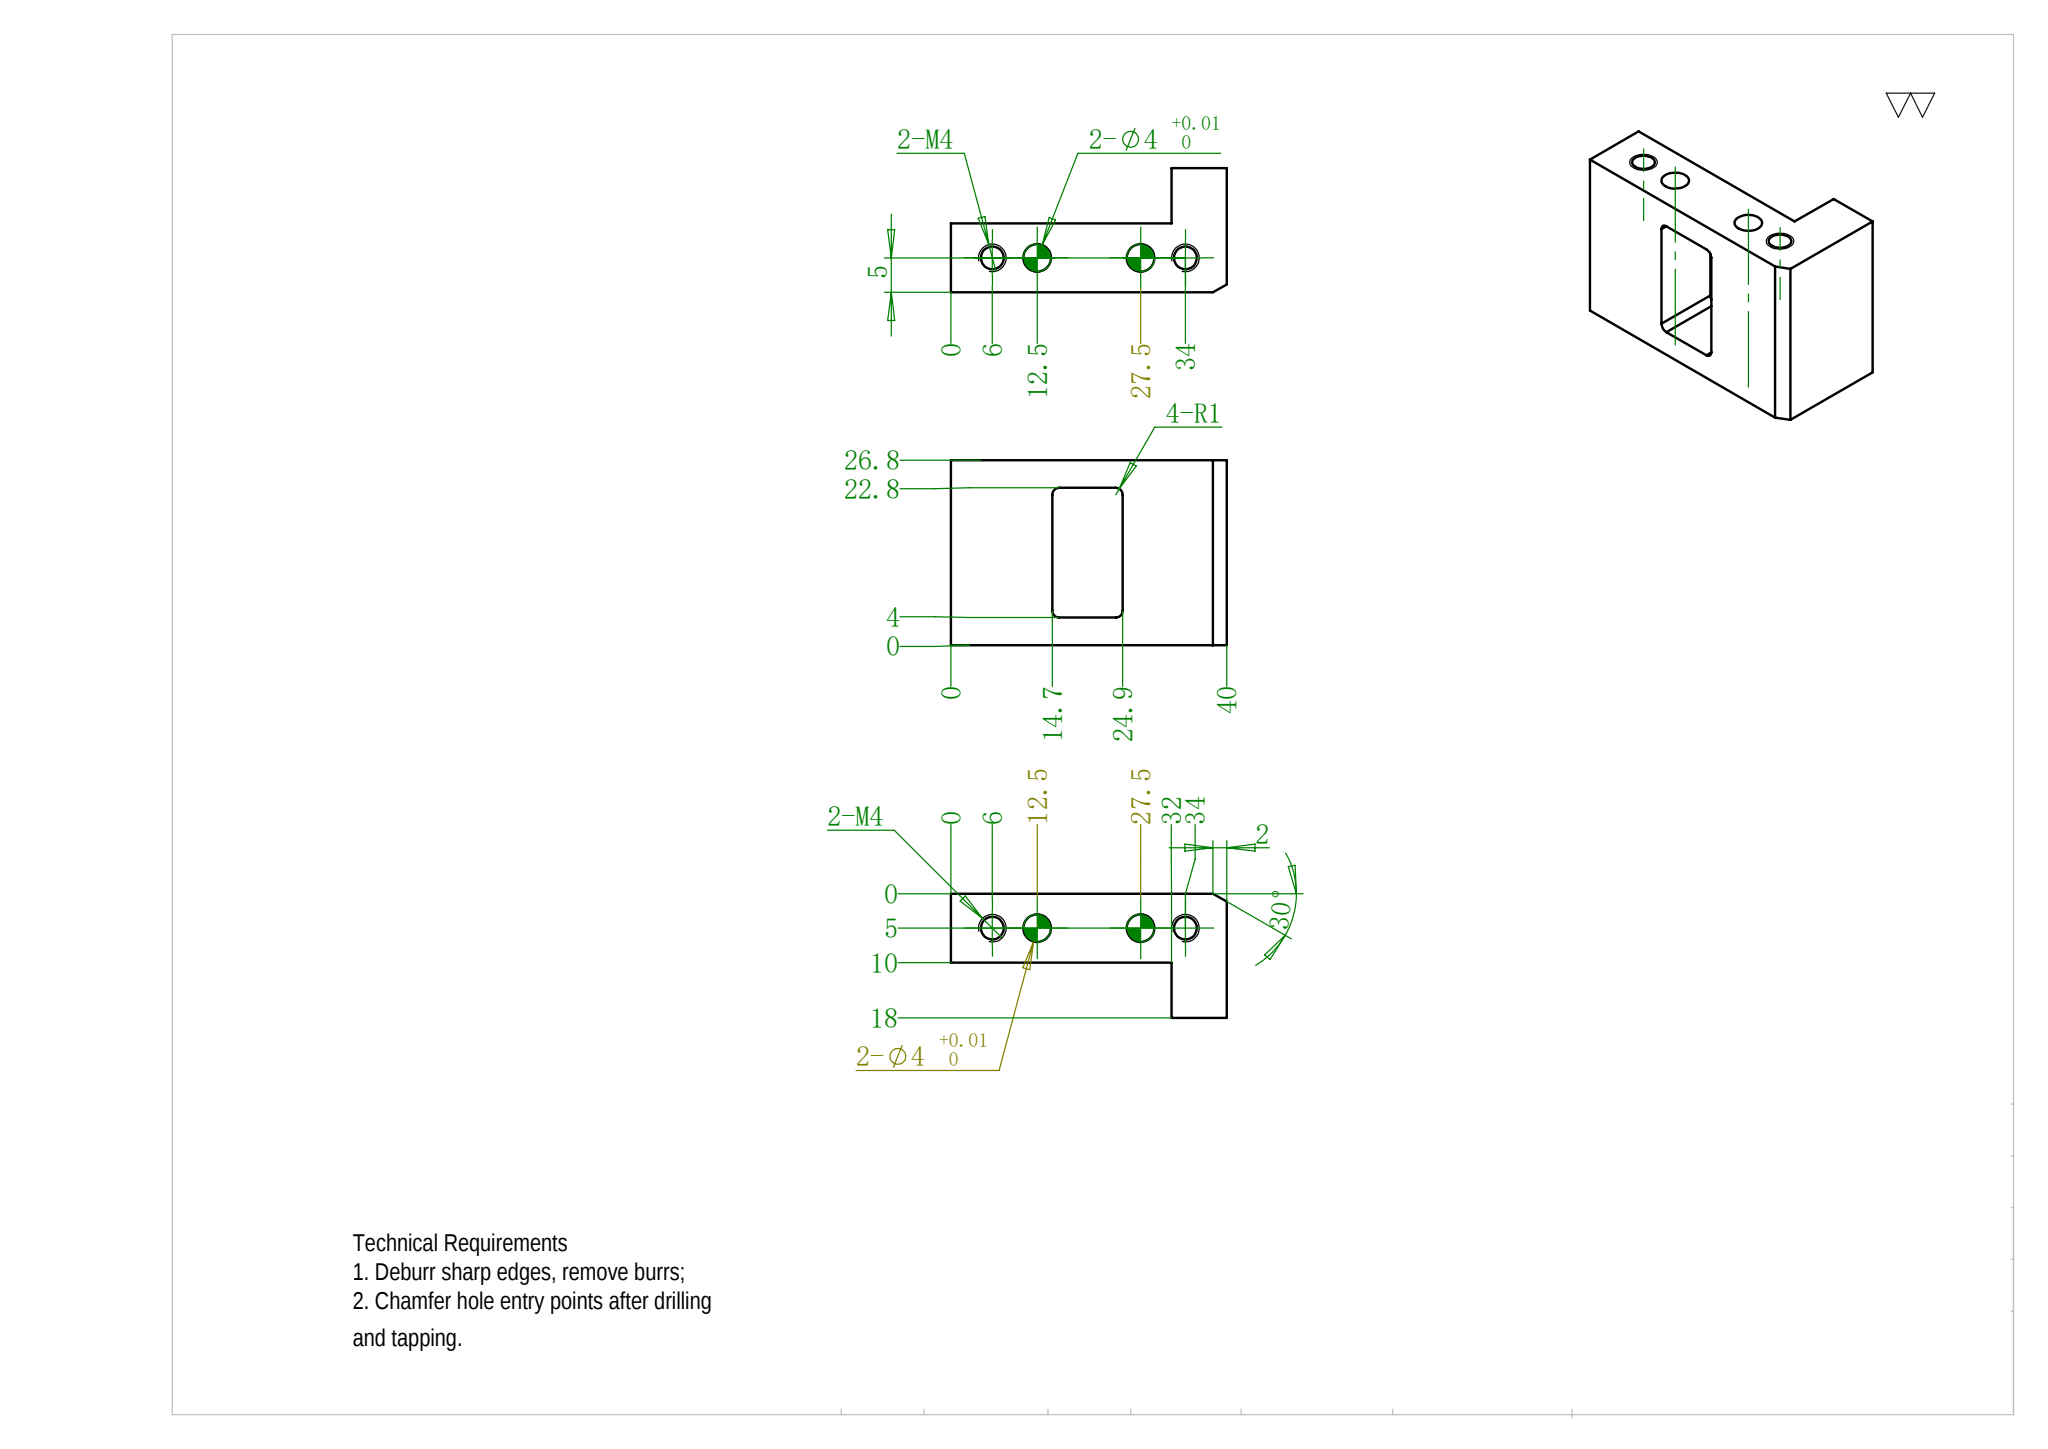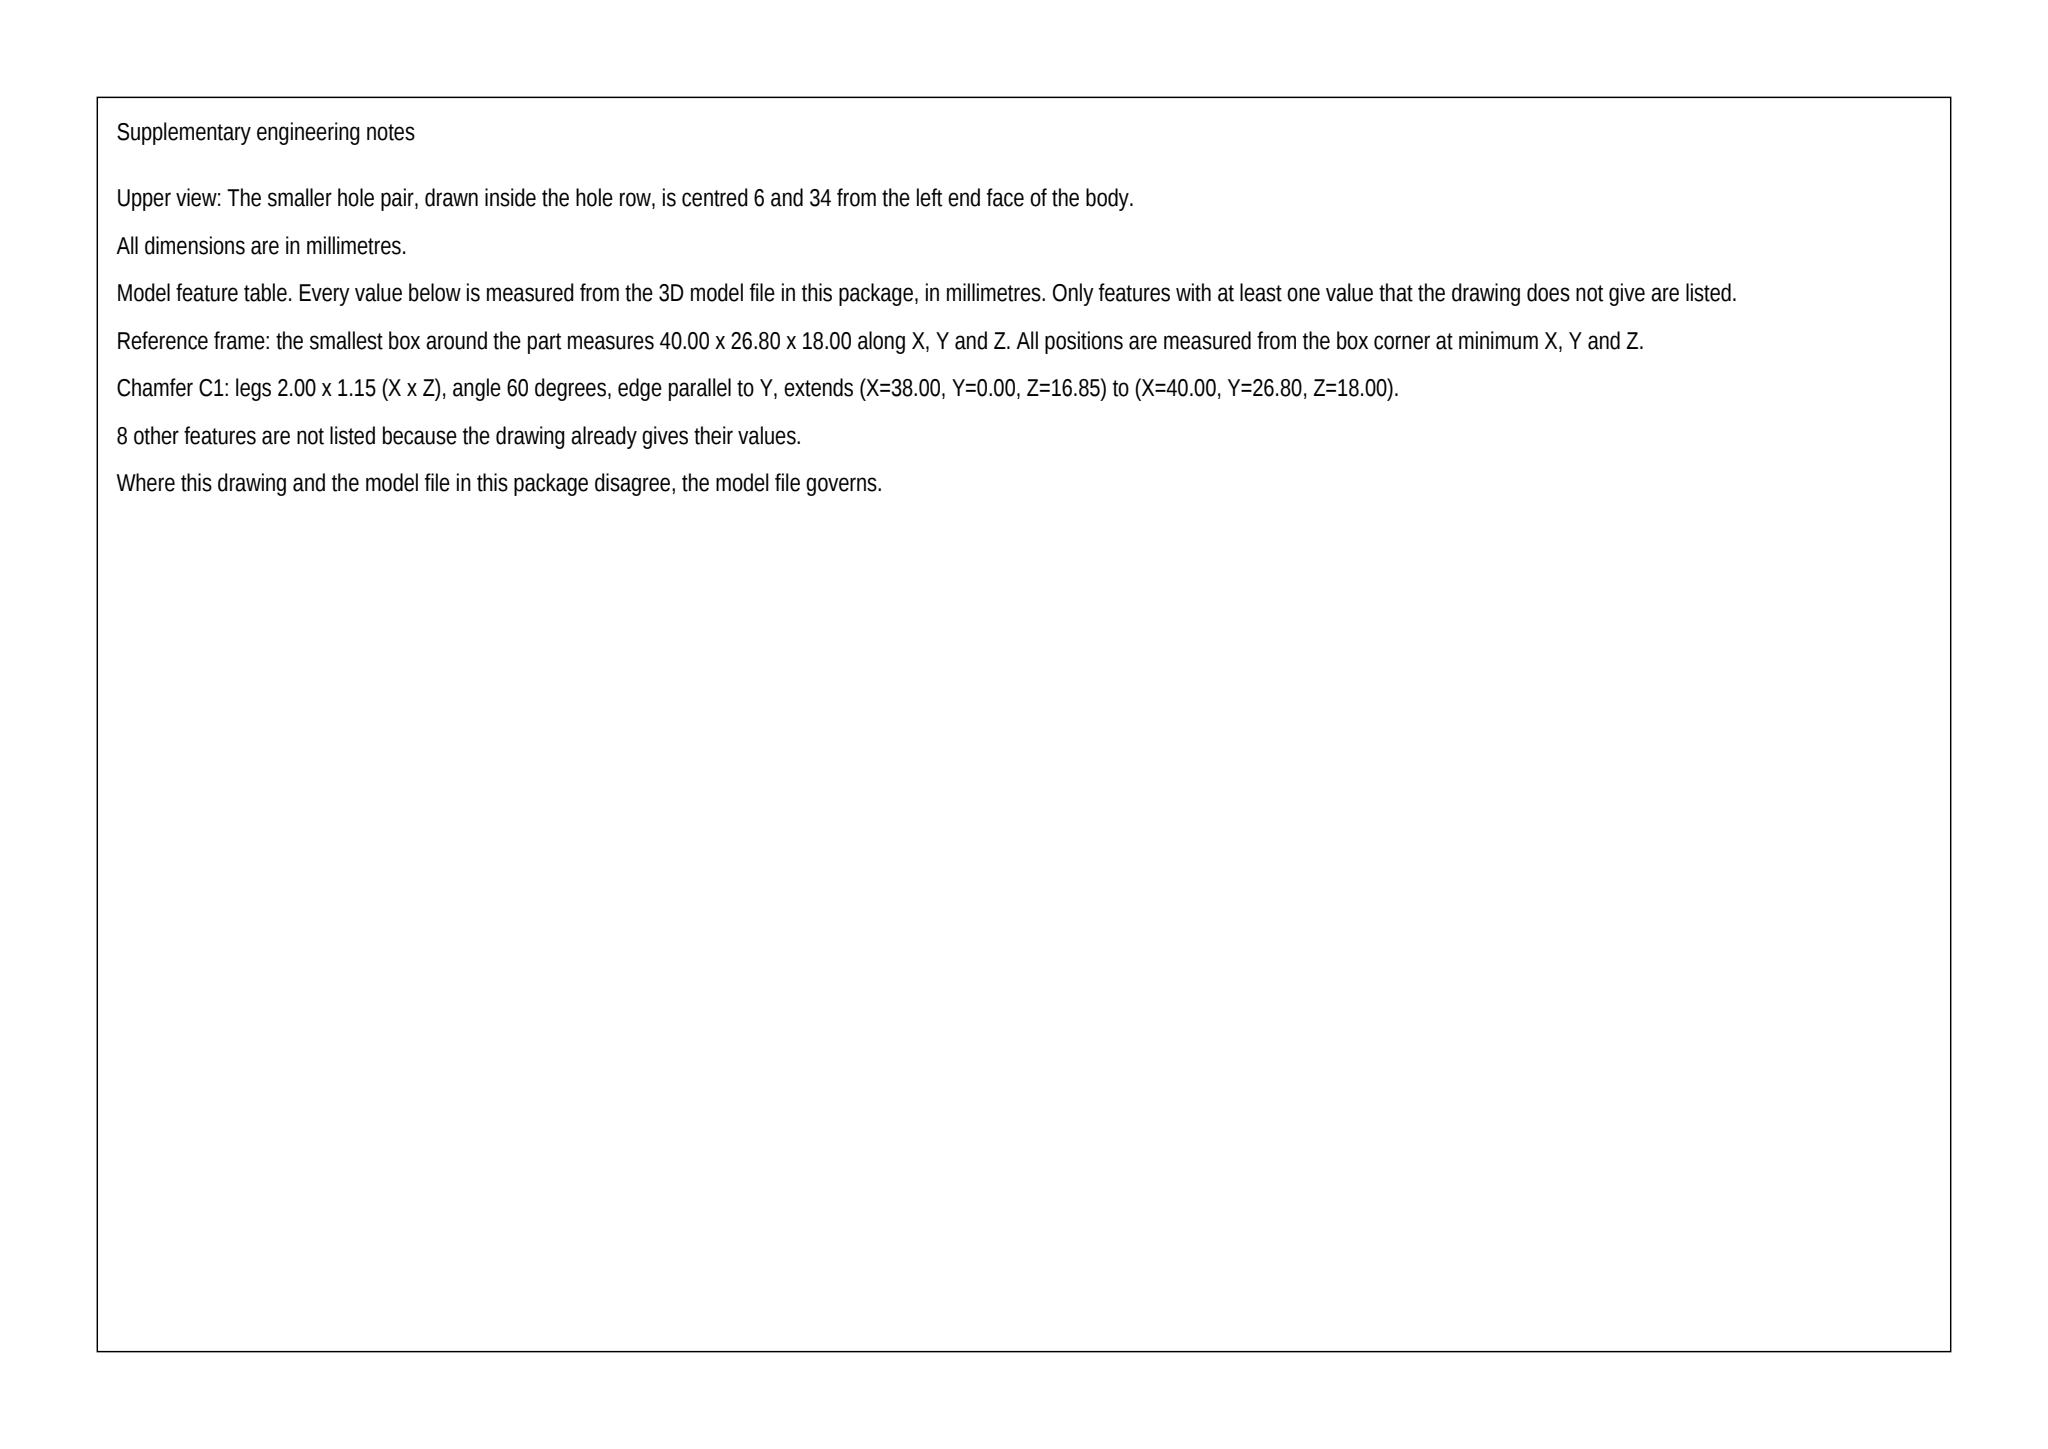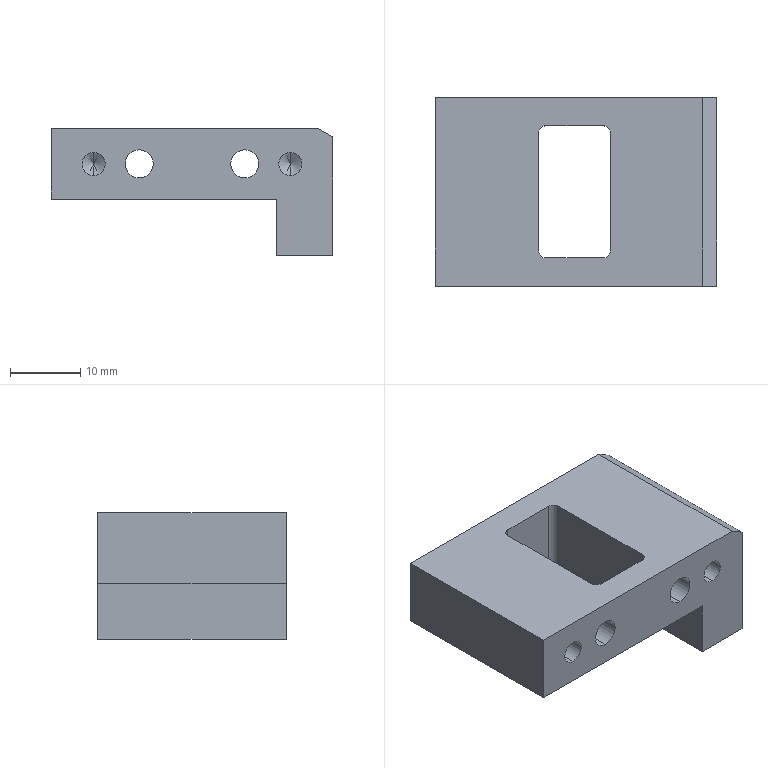Part | SolidWorks | mm | 1 solid | 37 faces | box 40 x 26.8 x 18 mm | volume 9537 mm3 | cylinder 16 | plane 13 | cone 8 | commonest cylinder face diameters 3.3 x8 4 x4 2 x4
build123d program:
from build123d import *

# Parameters (mm, degrees)
SKETCH1_W                  = 40
SKETCH1_H                  = 10
BOSS_EXTRUDE1_DEPTH        = 26.8
M4_TAPPED_HOLE1_AT_2_COUNT = 2
M4_TAPPED_HOLE1_AT_2_PITCH = 28
F_4_0_4_DIAMETER_HOLE1_D   = 4
SKETCH7_W                  = 8
SKETCH7_H                  = 26.8
BOSS_EXTRUDE2_DEPTH        = 8
SKETCH8_W                  = 10.2
SKETCH8_H                  = 18.8
CUT_EXTRUDE1_DEPTH         = 38.977
CHAMFER1_SIZE              = 2
CHAMFER1_SIZE2             = 1.155
FILLET1_R                  = 1


with BuildPart() as part:
    # Sketch1 → Boss-Extrude1 (new body)
    with BuildSketch(Plane(origin=(0, 0, 0), x_dir=(1, 0, 0), z_dir=(0, 1, 0))):
        Rectangle(SKETCH1_W, SKETCH1_H)
    extrude(amount=BOSS_EXTRUDE1_DEPTH)

    # Sketch3 → M4 Tapped Hole1 (revolve, cut)
    with BuildSketch(Plane(origin=(14, 26.8, 0), x_dir=(0, 0, 1), z_dir=(1, 0, 0))):
        Polygon((0, 0), (0, 8.991), (1.65, 8), (1.65, 0), align=None)
    m4_tapped_hole1 = revolve(axis=Axis((14, 33.15, 0), (0, -1, 0)), mode=Mode.SUBTRACT)

    # M4 Tapped Hole1 at 2: M4 Tapped Hole1 ×2
    with Locations(*[(-i * M4_TAPPED_HOLE1_AT_2_PITCH, 0, 0) for i in range(1, M4_TAPPED_HOLE1_AT_2_COUNT)]):
        add(m4_tapped_hole1, mode=Mode.SUBTRACT)

    # 4.0 _4_ Diameter Hole1 (through all)
    with Locations(Plane(origin=(0, 26.8, 0), x_dir=(1, 0, 0), z_dir=(0, 1, 0))):
        with Locations((7.5, 0), (-7.5, 0)):
            f_4_0_4_diameter_hole1 = Hole(F_4_0_4_DIAMETER_HOLE1_D / 2)

    # Mirror1: M4 Tapped Hole1, 4.0 _4_ Diameter Hole1 across plane
    add(m4_tapped_hole1.mirror(Plane.ZX.offset(13.4)), mode=Mode.SUBTRACT)
    add(f_4_0_4_diameter_hole1.mirror(Plane.ZX.offset(13.4)), mode=Mode.SUBTRACT)

    # Mirror1 copy 1 sketch → Mirror1 copy 1 (revolve, cut)
    with BuildSketch(Plane(origin=(-14, 0, 0), x_dir=(0, 0, 1), z_dir=(1, 0, 0))):
        Polygon((0, 0), (0, -8.991), (1.65, -8), (1.65, 0), align=None)
    revolve(axis=Axis((-14, -6.35, 0), (0, -1, 0)), mode=Mode.SUBTRACT)

    # Sketch7 → Boss-Extrude2 (add)
    with BuildSketch(Plane(origin=(0, 0, -5), x_dir=(-1, 0, 0), z_dir=(0, 0, -1))):
        with Locations((-16, 13.4)):
            Rectangle(SKETCH7_W, SKETCH7_H)
    extrude(amount=BOSS_EXTRUDE2_DEPTH)

    # Sketch8 → Cut-Extrude1 (cut, through all)
    with BuildSketch(Plane.XY.offset(5)):
        with Locations((-0.2, 13.4)):
            Rectangle(SKETCH8_W, SKETCH8_H)
    extrude(amount=-CUT_EXTRUDE1_DEPTH, mode=Mode.SUBTRACT)

    # Chamfer1
    chamfer1_edges = [part.edges().sort_by_distance(p)[0] for p in [
        (20, 13.4, 5),
    ]]
    chamfer1_side = [part.faces().sort_by_distance(p)[0] for p in [
        (19.519, 13.4, 5),
    ]]
    chamfer(chamfer1_edges, length=CHAMFER1_SIZE, length2=CHAMFER1_SIZE2, reference=chamfer1_side[0])

    # Fillet1
    fillet1_edges = [part.edges().sort_by_distance(p)[0] for p in [
        (-5.3, 4, 0),
        (-5.3, 22.8, 0),
        (4.9, 22.8, 0),
        (4.9, 4, 0),
    ]]
    fillet(fillet1_edges, radius=FILLET1_R)


solid = part.part